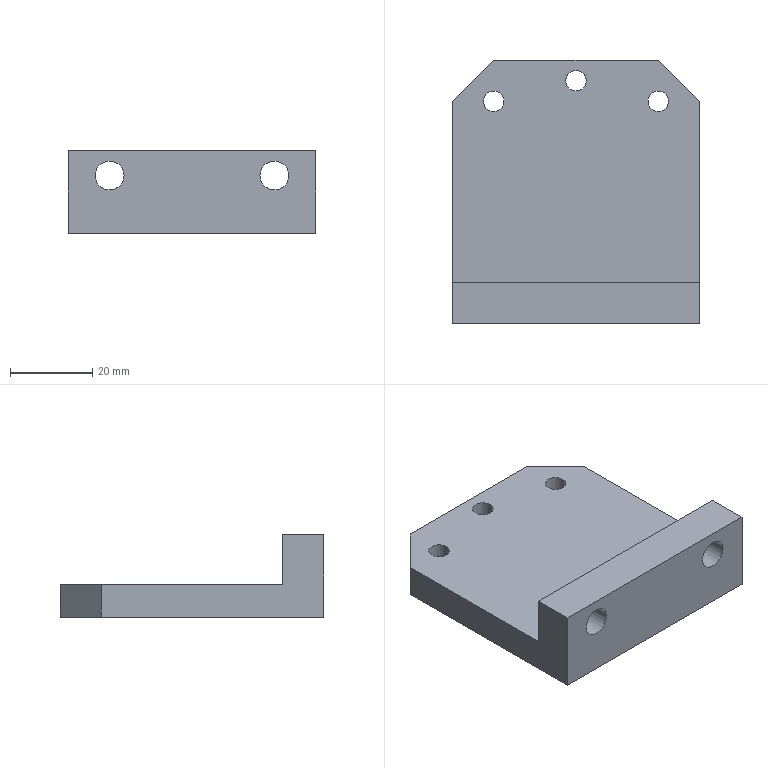Component | SolidWorks | STB-08-011-2 | 1 solid | 20 faces | box 60 x 64 x 20 mm | volume 35879 mm3 | cylinder 10 | plane 10 | commonest cylinder face diameters 5 x6 7 x4
build123d program:
from build123d import *

# Parameters (mm, degrees)
SKETCH1_W                = 20
SKETCH1_H                = 64
BOSS_EXTRUDE1_DEPTH      = 30
CUT_EXTRUDE1_REACH       = 70.731
SKETCH2_W                = 12
SKETCH2_H                = 54
M6_TAPPED_HOLE1_D        = 5
M6_TAPPED_HOLE2_D        = 5
M6_TAPPED_HOLE2_DEPTH    = 17
M6_TAPPED_HOLE2_TIP      = 1.502
CHAMFER1_SIZE            = 10
F_7_0_7_DIAMETER_HOLE1_D = 7


with BuildPart() as part:
    # Sketch1 → Boss-Extrude1 (new, symmetric)
    with BuildSketch(Plane.XY):
        Rectangle(SKETCH1_W, SKETCH1_H)
    extrude(amount=BOSS_EXTRUDE1_DEPTH, both=True)

    # Sketch2 → Cut-Extrude1 (cut, up to next)
    with BuildSketch(Plane.XY.offset(30), mode=Mode.PRIVATE) as cut_extrude1_sk1:
        with Locations((4, 5)):
            Rectangle(SKETCH2_W, SKETCH2_H)
    cut_extrude1_tool1 = extrude(cut_extrude1_sk1.sketch, amount=-CUT_EXTRUDE1_REACH, mode=Mode.PRIVATE) & part.part
    add(cut_extrude1_tool1.solids().sort_by_distance((4, 5, 30))[0], mode=Mode.SUBTRACT)

    # M6 Tapped Hole1 (through all)
    with Locations(Plane.ZY.offset(10)):
        with Locations((0, 27)):
            Hole(M6_TAPPED_HOLE1_D / 2)

    # M6 Tapped Hole2
    with Locations(Plane(origin=(-2, 0, 0), x_dir=(0, 0, -1), z_dir=(1, 0, 0))):
        with Locations((-20, 22), (20, 22)):
            Hole(M6_TAPPED_HOLE2_D / 2, depth=M6_TAPPED_HOLE2_DEPTH)
            with Locations((0, 0, -(M6_TAPPED_HOLE2_DEPTH + M6_TAPPED_HOLE2_TIP / 2))):  # 118° drill point
                Cone(0, M6_TAPPED_HOLE2_D / 2, M6_TAPPED_HOLE2_TIP, mode=Mode.SUBTRACT)

    # Chamfer1
    chamfer1_edges = [part.edges().sort_by_distance(p)[0] for p in [
        (-6, 32, -30),
        (-6, 32, 30),
    ]]
    chamfer(chamfer1_edges, length=CHAMFER1_SIZE)

    # 7.0 _7_ Diameter Hole1 (through all)
    with Locations(Plane(origin=(0, -22, 0), x_dir=(-1, 0, 0), z_dir=(0, 1, 0))):
        with Locations((-4, -20), (-4, 20)):
            Hole(F_7_0_7_DIAMETER_HOLE1_D / 2)


solid = part.part

# Placed as in the assembly
solid = solid.moved(Location((-104.904, 187.999, 11), (0, -90, 0)))
STEP:
#1=COLOUR_RGB('',0.7922,0.8196,0.9333);
#2=FILL_AREA_STYLE_COLOUR('',#1);
#3=FILL_AREA_STYLE('',(#2));
#4=SURFACE_STYLE_FILL_AREA(#3);
#5=SURFACE_SIDE_STYLE('',(#4));
#6=SURFACE_STYLE_USAGE(.BOTH.,#5);
#7=PRESENTATION_STYLE_ASSIGNMENT((#6));
#8=CARTESIAN_POINT('',(-3.205,6.142,0.5906));
#9=VERTEX_POINT('',#8);
#10=CARTESIAN_POINT('',(-3.48,6.142,0.5906));
#11=VERTEX_POINT('',#10);
#12=CARTESIAN_POINT('',(-3.343,6.142,0.5906));
#13=DIRECTION('',(-0.,1.,0.));
#14=DIRECTION('',(-1.,0.,0.));
#15=AXIS2_PLACEMENT_3D('',#12,#13,#14);
#16=CIRCLE('',#15,0.1378);
#17=EDGE_CURVE('',#9,#11,#16,.T.);
#18=ORIENTED_EDGE('',*,*,#17,.F.);
#19=CARTESIAN_POINT('',(-3.205,6.535,0.5906));
#20=VERTEX_POINT('',#19);
#21=CARTESIAN_POINT('',(-3.205,6.535,0.5906));
#22=DIRECTION('',(-0.,1.,0.));
#23=VECTOR('',#22,39.37);
#24=LINE('',#21,#23);
#25=EDGE_CURVE('',#9,#20,#24,.T.);
#26=ORIENTED_EDGE('',*,*,#25,.T.);
#27=CARTESIAN_POINT('',(-3.48,6.535,0.5906));
#28=VERTEX_POINT('',#27);
#29=CARTESIAN_POINT('',(-3.343,6.535,0.5906));
#30=DIRECTION('',(-0.,1.,0.));
#31=DIRECTION('',(-1.,0.,0.));
#32=AXIS2_PLACEMENT_3D('',#29,#30,#31);
#33=CIRCLE('',#32,0.1378);
#34=EDGE_CURVE('',#20,#28,#33,.T.);
#35=ORIENTED_EDGE('',*,*,#34,.T.);
#36=CARTESIAN_POINT('',(-3.48,6.535,0.5906));
#37=DIRECTION('',(-0.,1.,0.));
#38=VECTOR('',#37,39.37);
#39=LINE('',#36,#38);
#40=EDGE_CURVE('',#11,#28,#39,.T.);
#41=ORIENTED_EDGE('',*,*,#40,.F.);
#42=EDGE_LOOP('',(#18,#26,#35,#41));
#43=FACE_OUTER_BOUND('',#42,.T.);
#44=CARTESIAN_POINT('',(-3.343,6.535,0.5906));
#45=DIRECTION('',(-0.,1.,0.));
#46=DIRECTION('',(-1.,0.,0.));
#47=AXIS2_PLACEMENT_3D('',#44,#45,#46);
#48=CYLINDRICAL_SURFACE('',#47,0.1378);
#49=ADVANCED_FACE('',(#43),#48,.F.);
#50=CARTESIAN_POINT('',(-4.78,6.142,0.5906));
#51=VERTEX_POINT('',#50);
#52=CARTESIAN_POINT('',(-5.055,6.142,0.5906));
#53=VERTEX_POINT('',#52);
#54=CARTESIAN_POINT('',(-4.917,6.142,0.5906));
#55=DIRECTION('',(-0.,1.,0.));
#56=DIRECTION('',(-1.,0.,0.));
#57=AXIS2_PLACEMENT_3D('',#54,#55,#56);
#58=CIRCLE('',#57,0.1378);
#59=EDGE_CURVE('',#51,#53,#58,.T.);
#60=ORIENTED_EDGE('',*,*,#59,.F.);
#61=CARTESIAN_POINT('',(-4.78,6.535,0.5906));
#62=VERTEX_POINT('',#61);
#63=CARTESIAN_POINT('',(-4.78,6.535,0.5906));
#64=DIRECTION('',(-0.,1.,0.));
#65=VECTOR('',#64,39.37);
#66=LINE('',#63,#65);
#67=EDGE_CURVE('',#51,#62,#66,.T.);
#68=ORIENTED_EDGE('',*,*,#67,.T.);
#69=CARTESIAN_POINT('',(-5.055,6.535,0.5906));
#70=VERTEX_POINT('',#69);
#71=CARTESIAN_POINT('',(-4.917,6.535,0.5906));
#72=DIRECTION('',(-0.,1.,0.));
#73=DIRECTION('',(-1.,0.,0.));
#74=AXIS2_PLACEMENT_3D('',#71,#72,#73);
#75=CIRCLE('',#74,0.1378);
#76=EDGE_CURVE('',#62,#70,#75,.T.);
#77=ORIENTED_EDGE('',*,*,#76,.T.);
#78=CARTESIAN_POINT('',(-5.055,6.535,0.5906));
#79=DIRECTION('',(-0.,1.,0.));
#80=VECTOR('',#79,39.37);
#81=LINE('',#78,#80);
#82=EDGE_CURVE('',#53,#70,#81,.T.);
#83=ORIENTED_EDGE('',*,*,#82,.F.);
#84=EDGE_LOOP('',(#60,#68,#77,#83));
#85=FACE_OUTER_BOUND('',#84,.T.);
#86=CARTESIAN_POINT('',(-4.917,6.535,0.5906));
#87=DIRECTION('',(-0.,1.,0.));
#88=DIRECTION('',(-1.,0.,0.));
#89=AXIS2_PLACEMENT_3D('',#86,#87,#88);
#90=CYLINDRICAL_SURFACE('',#89,0.1378);
#91=ADVANCED_FACE('',(#85),#90,.F.);
#92=CARTESIAN_POINT('',(-5.016,8.268,0.03937));
#93=VERTEX_POINT('',#92);
#94=CARTESIAN_POINT('',(-4.819,8.268,0.03937));
#95=VERTEX_POINT('',#94);
#96=CARTESIAN_POINT('',(-4.917,8.268,0.03937));
#97=DIRECTION('',(-0.,0.,1.));
#98=DIRECTION('',(1.,0.,0.));
#99=AXIS2_PLACEMENT_3D('',#96,#97,#98);
#100=CIRCLE('',#99,0.09843);
#101=EDGE_CURVE('',#93,#95,#100,.T.);
#102=ORIENTED_EDGE('',*,*,#101,.F.);
#103=CARTESIAN_POINT('',(-5.016,8.268,0.3543));
#104=VERTEX_POINT('',#103);
#105=CARTESIAN_POINT('',(-5.016,8.268,0.3543));
#106=DIRECTION('',(-0.,0.,1.));
#107=VECTOR('',#106,39.37);
#108=LINE('',#105,#107);
#109=EDGE_CURVE('',#93,#104,#108,.T.);
#110=ORIENTED_EDGE('',*,*,#109,.T.);
#111=CARTESIAN_POINT('',(-4.819,8.268,0.3543));
#112=VERTEX_POINT('',#111);
#113=CARTESIAN_POINT('',(-4.917,8.268,0.3543));
#114=DIRECTION('',(-0.,0.,1.));
#115=DIRECTION('',(1.,0.,0.));
#116=AXIS2_PLACEMENT_3D('',#113,#114,#115);
#117=CIRCLE('',#116,0.09843);
#118=EDGE_CURVE('',#104,#112,#117,.T.);
#119=ORIENTED_EDGE('',*,*,#118,.T.);
#120=CARTESIAN_POINT('',(-4.819,8.268,0.3543));
#121=DIRECTION('',(-0.,0.,1.));
#122=VECTOR('',#121,39.37);
#123=LINE('',#120,#122);
#124=EDGE_CURVE('',#95,#112,#123,.T.);
#125=ORIENTED_EDGE('',*,*,#124,.F.);
#126=EDGE_LOOP('',(#102,#110,#119,#125));
#127=FACE_OUTER_BOUND('',#126,.T.);
#128=CARTESIAN_POINT('',(-4.917,8.268,0.3543));
#129=DIRECTION('',(-0.,0.,1.));
#130=DIRECTION('',(1.,0.,0.));
#131=AXIS2_PLACEMENT_3D('',#128,#129,#130);
#132=CYLINDRICAL_SURFACE('',#131,0.09843);
#133=ADVANCED_FACE('',(#127),#132,.F.);
#134=CARTESIAN_POINT('',(-3.441,8.268,0.03937));
#135=VERTEX_POINT('',#134);
#136=CARTESIAN_POINT('',(-3.244,8.268,0.03937));
#137=VERTEX_POINT('',#136);
#138=CARTESIAN_POINT('',(-3.343,8.268,0.03937));
#139=DIRECTION('',(-0.,0.,1.));
#140=DIRECTION('',(1.,0.,0.));
#141=AXIS2_PLACEMENT_3D('',#138,#139,#140);
#142=CIRCLE('',#141,0.09843);
#143=EDGE_CURVE('',#135,#137,#142,.T.);
#144=ORIENTED_EDGE('',*,*,#143,.F.);
#145=CARTESIAN_POINT('',(-3.441,8.268,0.3543));
#146=VERTEX_POINT('',#145);
#147=CARTESIAN_POINT('',(-3.441,8.268,0.3543));
#148=DIRECTION('',(-0.,0.,1.));
#149=VECTOR('',#148,39.37);
#150=LINE('',#147,#149);
#151=EDGE_CURVE('',#135,#146,#150,.T.);
#152=ORIENTED_EDGE('',*,*,#151,.T.);
#153=CARTESIAN_POINT('',(-3.244,8.268,0.3543));
#154=VERTEX_POINT('',#153);
#155=CARTESIAN_POINT('',(-3.343,8.268,0.3543));
#156=DIRECTION('',(-0.,0.,1.));
#157=DIRECTION('',(1.,0.,0.));
#158=AXIS2_PLACEMENT_3D('',#155,#156,#157);
#159=CIRCLE('',#158,0.09843);
#160=EDGE_CURVE('',#146,#154,#159,.T.);
#161=ORIENTED_EDGE('',*,*,#160,.T.);
#162=CARTESIAN_POINT('',(-3.244,8.268,0.3543));
#163=DIRECTION('',(-0.,0.,1.));
#164=VECTOR('',#163,39.37);
#165=LINE('',#162,#164);
#166=EDGE_CURVE('',#137,#154,#165,.T.);
#167=ORIENTED_EDGE('',*,*,#166,.F.);
#168=EDGE_LOOP('',(#144,#152,#161,#167));
#169=FACE_OUTER_BOUND('',#168,.T.);
#170=CARTESIAN_POINT('',(-3.343,8.268,0.3543));
#171=DIRECTION('',(-0.,0.,1.));
#172=DIRECTION('',(1.,0.,0.));
#173=AXIS2_PLACEMENT_3D('',#170,#171,#172);
#174=CYLINDRICAL_SURFACE('',#173,0.09843);
#175=ADVANCED_FACE('',(#169),#174,.F.);
#176=CARTESIAN_POINT('',(-4.032,8.465,0.3543));
#177=VERTEX_POINT('',#176);
#178=CARTESIAN_POINT('',(-4.228,8.465,0.3543));
#179=VERTEX_POINT('',#178);
#180=CARTESIAN_POINT('',(-4.13,8.465,0.3543));
#181=DIRECTION('',(0.,-0.,-1.));
#182=DIRECTION('',(0.,-1.,0.));
#183=AXIS2_PLACEMENT_3D('',#180,#181,#182);
#184=CIRCLE('',#183,0.09843);
#185=EDGE_CURVE('',#177,#179,#184,.T.);
#186=ORIENTED_EDGE('',*,*,#185,.F.);
#187=CARTESIAN_POINT('',(-4.032,8.465,0.03937));
#188=VERTEX_POINT('',#187);
#189=CARTESIAN_POINT('',(-4.032,8.465,0.03937));
#190=DIRECTION('',(0.,-0.,-1.));
#191=VECTOR('',#190,39.37);
#192=LINE('',#189,#191);
#193=EDGE_CURVE('',#177,#188,#192,.T.);
#194=ORIENTED_EDGE('',*,*,#193,.T.);
#195=CARTESIAN_POINT('',(-4.228,8.465,0.03937));
#196=VERTEX_POINT('',#195);
#197=CARTESIAN_POINT('',(-4.13,8.465,0.03937));
#198=DIRECTION('',(0.,-0.,-1.));
#199=DIRECTION('',(-1.,0.,-0.));
#200=AXIS2_PLACEMENT_3D('',#197,#198,#199);
#201=CIRCLE('',#200,0.09843);
#202=EDGE_CURVE('',#188,#196,#201,.T.);
#203=ORIENTED_EDGE('',*,*,#202,.T.);
#204=CARTESIAN_POINT('',(-4.228,8.465,0.03937));
#205=DIRECTION('',(0.,-0.,-1.));
#206=VECTOR('',#205,39.37);
#207=LINE('',#204,#206);
#208=EDGE_CURVE('',#179,#196,#207,.T.);
#209=ORIENTED_EDGE('',*,*,#208,.F.);
#210=EDGE_LOOP('',(#186,#194,#203,#209));
#211=FACE_OUTER_BOUND('',#210,.T.);
#212=CARTESIAN_POINT('',(-4.13,8.465,0.03937));
#213=DIRECTION('',(0.,-0.,-1.));
#214=DIRECTION('',(-1.,0.,-0.));
#215=AXIS2_PLACEMENT_3D('',#212,#213,#214);
#216=CYLINDRICAL_SURFACE('',#215,0.09843);
#217=ADVANCED_FACE('',(#211),#216,.F.);
#218=CARTESIAN_POINT('',(-4.13,8.465,0.3543));
#219=DIRECTION('',(0.,-0.,-1.));
#220=DIRECTION('',(0.,-1.,0.));
#221=AXIS2_PLACEMENT_3D('',#218,#219,#220);
#222=CIRCLE('',#221,0.09843);
#223=EDGE_CURVE('',#179,#177,#222,.T.);
#224=ORIENTED_EDGE('',*,*,#223,.T.);
#225=ORIENTED_EDGE('',*,*,#185,.T.);
#226=EDGE_LOOP('',(#224,#225));
#227=FACE_BOUND('',#226,.T.);
#228=CARTESIAN_POINT('',(-2.949,6.535,0.3543));
#229=VERTEX_POINT('',#228);
#230=CARTESIAN_POINT('',(-2.949,8.268,0.3543));
#231=VERTEX_POINT('',#230);
#232=CARTESIAN_POINT('',(-2.949,8.661,0.3543));
#233=DIRECTION('',(-0.,1.,-0.));
#234=VECTOR('',#233,39.37);
#235=LINE('',#232,#234);
#236=EDGE_CURVE('',#229,#231,#235,.T.);
#237=ORIENTED_EDGE('',*,*,#236,.T.);
#238=CARTESIAN_POINT('',(-3.343,8.661,0.3543));
#239=VERTEX_POINT('',#238);
#240=CARTESIAN_POINT('',(-3.343,8.661,0.3543));
#241=DIRECTION('',(-0.7071,0.7071,-0.));
#242=VECTOR('',#241,39.37);
#243=LINE('',#240,#242);
#244=EDGE_CURVE('',#231,#239,#243,.T.);
#245=ORIENTED_EDGE('',*,*,#244,.T.);
#246=CARTESIAN_POINT('',(-4.917,8.661,0.3543));
#247=VERTEX_POINT('',#246);
#248=CARTESIAN_POINT('',(-2.949,8.661,0.3543));
#249=DIRECTION('',(-1.,0.,-0.));
#250=VECTOR('',#249,39.37);
#251=LINE('',#248,#250);
#252=EDGE_CURVE('',#239,#247,#251,.T.);
#253=ORIENTED_EDGE('',*,*,#252,.T.);
#254=CARTESIAN_POINT('',(-5.311,8.268,0.3543));
#255=VERTEX_POINT('',#254);
#256=CARTESIAN_POINT('',(-5.311,8.268,0.3543));
#257=DIRECTION('',(-0.7071,-0.7071,-0.));
#258=VECTOR('',#257,39.37);
#259=LINE('',#256,#258);
#260=EDGE_CURVE('',#247,#255,#259,.T.);
#261=ORIENTED_EDGE('',*,*,#260,.T.);
#262=CARTESIAN_POINT('',(-5.311,6.535,0.3543));
#263=VERTEX_POINT('',#262);
#264=CARTESIAN_POINT('',(-5.311,8.661,0.3543));
#265=DIRECTION('',(0.,-1.,0.));
#266=VECTOR('',#265,39.37);
#267=LINE('',#264,#266);
#268=EDGE_CURVE('',#255,#263,#267,.T.);
#269=ORIENTED_EDGE('',*,*,#268,.T.);
#270=CARTESIAN_POINT('',(-2.949,6.535,0.3543));
#271=DIRECTION('',(-1.,0.,-0.));
#272=VECTOR('',#271,39.37);
#273=LINE('',#270,#272);
#274=EDGE_CURVE('',#229,#263,#273,.T.);
#275=ORIENTED_EDGE('',*,*,#274,.F.);
#276=EDGE_LOOP('',(#237,#245,#253,#261,#269,#275));
#277=FACE_OUTER_BOUND('',#276,.T.);
#278=CARTESIAN_POINT('',(-3.343,8.268,0.3543));
#279=DIRECTION('',(-0.,0.,1.));
#280=DIRECTION('',(1.,0.,0.));
#281=AXIS2_PLACEMENT_3D('',#278,#279,#280);
#282=CIRCLE('',#281,0.09843);
#283=EDGE_CURVE('',#154,#146,#282,.T.);
#284=ORIENTED_EDGE('',*,*,#283,.F.);
#285=ORIENTED_EDGE('',*,*,#160,.F.);
#286=EDGE_LOOP('',(#284,#285));
#287=FACE_BOUND('',#286,.T.);
#288=CARTESIAN_POINT('',(-4.917,8.268,0.3543));
#289=DIRECTION('',(-0.,0.,1.));
#290=DIRECTION('',(1.,0.,0.));
#291=AXIS2_PLACEMENT_3D('',#288,#289,#290);
#292=CIRCLE('',#291,0.09843);
#293=EDGE_CURVE('',#112,#104,#292,.T.);
#294=ORIENTED_EDGE('',*,*,#293,.F.);
#295=ORIENTED_EDGE('',*,*,#118,.F.);
#296=EDGE_LOOP('',(#294,#295));
#297=FACE_BOUND('',#296,.T.);
#298=CARTESIAN_POINT('',(-2.949,8.661,0.3543));
#299=DIRECTION('',(0.,-0.,-1.));
#300=DIRECTION('',(0.,-1.,0.));
#301=AXIS2_PLACEMENT_3D('',#298,#299,#300);
#302=PLANE('',#301);
#303=ADVANCED_FACE('',(#227,#277,#287,#297),#302,.F.);
#304=CARTESIAN_POINT('',(-4.917,8.268,0.03937));
#305=DIRECTION('',(-0.,0.,1.));
#306=DIRECTION('',(1.,0.,0.));
#307=AXIS2_PLACEMENT_3D('',#304,#305,#306);
#308=CIRCLE('',#307,0.09843);
#309=EDGE_CURVE('',#95,#93,#308,.T.);
#310=ORIENTED_EDGE('',*,*,#309,.T.);
#311=ORIENTED_EDGE('',*,*,#101,.T.);
#312=EDGE_LOOP('',(#310,#311));
#313=FACE_BOUND('',#312,.T.);
#314=CARTESIAN_POINT('',(-3.343,8.268,0.03937));
#315=DIRECTION('',(-0.,0.,1.));
#316=DIRECTION('',(1.,0.,0.));
#317=AXIS2_PLACEMENT_3D('',#314,#315,#316);
#318=CIRCLE('',#317,0.09843);
#319=EDGE_CURVE('',#137,#135,#318,.T.);
#320=ORIENTED_EDGE('',*,*,#319,.T.);
#321=ORIENTED_EDGE('',*,*,#143,.T.);
#322=EDGE_LOOP('',(#320,#321));
#323=FACE_BOUND('',#322,.T.);
#324=CARTESIAN_POINT('',(-4.13,8.465,0.03937));
#325=DIRECTION('',(0.,-0.,-1.));
#326=DIRECTION('',(-1.,0.,-0.));
#327=AXIS2_PLACEMENT_3D('',#324,#325,#326);
#328=CIRCLE('',#327,0.09843);
#329=EDGE_CURVE('',#196,#188,#328,.T.);
#330=ORIENTED_EDGE('',*,*,#329,.F.);
#331=ORIENTED_EDGE('',*,*,#202,.F.);
#332=EDGE_LOOP('',(#330,#331));
#333=FACE_BOUND('',#332,.T.);
#334=CARTESIAN_POINT('',(-4.917,8.661,0.03937));
#335=VERTEX_POINT('',#334);
#336=CARTESIAN_POINT('',(-3.343,8.661,0.03937));
#337=VERTEX_POINT('',#336);
#338=CARTESIAN_POINT('',(-5.311,8.661,0.03937));
#339=DIRECTION('',(1.,-0.,0.));
#340=VECTOR('',#339,39.37);
#341=LINE('',#338,#340);
#342=EDGE_CURVE('',#335,#337,#341,.T.);
#343=ORIENTED_EDGE('',*,*,#342,.T.);
#344=CARTESIAN_POINT('',(-2.949,8.268,0.03937));
#345=VERTEX_POINT('',#344);
#346=CARTESIAN_POINT('',(-3.343,8.661,0.03937));
#347=DIRECTION('',(0.7071,-0.7071,0.));
#348=VECTOR('',#347,39.37);
#349=LINE('',#346,#348);
#350=EDGE_CURVE('',#337,#345,#349,.T.);
#351=ORIENTED_EDGE('',*,*,#350,.T.);
#352=CARTESIAN_POINT('',(-2.949,6.142,0.03937));
#353=VERTEX_POINT('',#352);
#354=CARTESIAN_POINT('',(-2.949,8.661,0.03937));
#355=DIRECTION('',(0.,-1.,-0.));
#356=VECTOR('',#355,39.37);
#357=LINE('',#354,#356);
#358=EDGE_CURVE('',#345,#353,#357,.T.);
#359=ORIENTED_EDGE('',*,*,#358,.T.);
#360=CARTESIAN_POINT('',(-5.311,6.142,0.03937));
#361=VERTEX_POINT('',#360);
#362=CARTESIAN_POINT('',(-5.311,6.142,0.03937));
#363=DIRECTION('',(1.,-0.,0.));
#364=VECTOR('',#363,39.37);
#365=LINE('',#362,#364);
#366=EDGE_CURVE('',#361,#353,#365,.T.);
#367=ORIENTED_EDGE('',*,*,#366,.F.);
#368=CARTESIAN_POINT('',(-5.311,8.268,0.03937));
#369=VERTEX_POINT('',#368);
#370=CARTESIAN_POINT('',(-5.311,8.661,0.03937));
#371=DIRECTION('',(0.,-1.,-0.));
#372=VECTOR('',#371,39.37);
#373=LINE('',#370,#372);
#374=EDGE_CURVE('',#369,#361,#373,.T.);
#375=ORIENTED_EDGE('',*,*,#374,.F.);
#376=CARTESIAN_POINT('',(-5.311,8.268,0.03937));
#377=DIRECTION('',(0.7071,0.7071,0.));
#378=VECTOR('',#377,39.37);
#379=LINE('',#376,#378);
#380=EDGE_CURVE('',#369,#335,#379,.T.);
#381=ORIENTED_EDGE('',*,*,#380,.T.);
#382=EDGE_LOOP('',(#343,#351,#359,#367,#375,#381));
#383=FACE_OUTER_BOUND('',#382,.T.);
#384=CARTESIAN_POINT('',(-5.311,8.661,0.03937));
#385=DIRECTION('',(-0.,0.,1.));
#386=DIRECTION('',(1.,-0.,0.));
#387=AXIS2_PLACEMENT_3D('',#384,#385,#386);
#388=PLANE('',#387);
#389=ADVANCED_FACE('',(#313,#323,#333,#383),#388,.F.);
#390=CARTESIAN_POINT('',(-3.343,6.142,0.5906));
#391=DIRECTION('',(-0.,1.,0.));
#392=DIRECTION('',(-1.,0.,0.));
#393=AXIS2_PLACEMENT_3D('',#390,#391,#392);
#394=CIRCLE('',#393,0.1378);
#395=EDGE_CURVE('',#11,#9,#394,.T.);
#396=ORIENTED_EDGE('',*,*,#395,.T.);
#397=ORIENTED_EDGE('',*,*,#17,.T.);
#398=EDGE_LOOP('',(#396,#397));
#399=FACE_BOUND('',#398,.T.);
#400=CARTESIAN_POINT('',(-4.917,6.142,0.5906));
#401=DIRECTION('',(-0.,1.,0.));
#402=DIRECTION('',(-1.,0.,0.));
#403=AXIS2_PLACEMENT_3D('',#400,#401,#402);
#404=CIRCLE('',#403,0.1378);
#405=EDGE_CURVE('',#53,#51,#404,.T.);
#406=ORIENTED_EDGE('',*,*,#405,.T.);
#407=ORIENTED_EDGE('',*,*,#59,.T.);
#408=EDGE_LOOP('',(#406,#407));
#409=FACE_BOUND('',#408,.T.);
#410=CARTESIAN_POINT('',(-2.949,6.142,0.8268));
#411=VERTEX_POINT('',#410);
#412=CARTESIAN_POINT('',(-2.949,6.142,0.03937));
#413=DIRECTION('',(-0.,0.,1.));
#414=VECTOR('',#413,39.37);
#415=LINE('',#412,#414);
#416=EDGE_CURVE('',#353,#411,#415,.T.);
#417=ORIENTED_EDGE('',*,*,#416,.T.);
#418=CARTESIAN_POINT('',(-5.311,6.142,0.8268));
#419=VERTEX_POINT('',#418);
#420=CARTESIAN_POINT('',(-5.311,6.142,0.8268));
#421=DIRECTION('',(1.,-0.,0.));
#422=VECTOR('',#421,39.37);
#423=LINE('',#420,#422);
#424=EDGE_CURVE('',#419,#411,#423,.T.);
#425=ORIENTED_EDGE('',*,*,#424,.F.);
#426=CARTESIAN_POINT('',(-5.311,6.142,0.03937));
#427=DIRECTION('',(-0.,0.,1.));
#428=VECTOR('',#427,39.37);
#429=LINE('',#426,#428);
#430=EDGE_CURVE('',#361,#419,#429,.T.);
#431=ORIENTED_EDGE('',*,*,#430,.F.);
#432=ORIENTED_EDGE('',*,*,#366,.T.);
#433=EDGE_LOOP('',(#417,#425,#431,#432));
#434=FACE_OUTER_BOUND('',#433,.T.);
#435=CARTESIAN_POINT('',(-5.311,6.142,0.03937));
#436=DIRECTION('',(0.,1.,0.));
#437=DIRECTION('',(-1.,0.,-0.));
#438=AXIS2_PLACEMENT_3D('',#435,#436,#437);
#439=PLANE('',#438);
#440=ADVANCED_FACE('',(#399,#409,#434),#439,.F.);
#441=CARTESIAN_POINT('',(-2.949,6.535,0.8268));
#442=VERTEX_POINT('',#441);
#443=CARTESIAN_POINT('',(-2.949,8.661,0.8268));
#444=DIRECTION('',(-0.,1.,0.));
#445=VECTOR('',#444,39.37);
#446=LINE('',#443,#445);
#447=EDGE_CURVE('',#411,#442,#446,.T.);
#448=ORIENTED_EDGE('',*,*,#447,.T.);
#449=CARTESIAN_POINT('',(-5.311,6.535,0.8268));
#450=VERTEX_POINT('',#449);
#451=CARTESIAN_POINT('',(-2.949,6.535,0.8268));
#452=DIRECTION('',(-1.,0.,-0.));
#453=VECTOR('',#452,39.37);
#454=LINE('',#451,#453);
#455=EDGE_CURVE('',#442,#450,#454,.T.);
#456=ORIENTED_EDGE('',*,*,#455,.T.);
#457=CARTESIAN_POINT('',(-5.311,8.661,0.8268));
#458=DIRECTION('',(-0.,1.,0.));
#459=VECTOR('',#458,39.37);
#460=LINE('',#457,#459);
#461=EDGE_CURVE('',#419,#450,#460,.T.);
#462=ORIENTED_EDGE('',*,*,#461,.F.);
#463=ORIENTED_EDGE('',*,*,#424,.T.);
#464=EDGE_LOOP('',(#448,#456,#462,#463));
#465=FACE_OUTER_BOUND('',#464,.T.);
#466=CARTESIAN_POINT('',(-5.311,8.661,0.8268));
#467=DIRECTION('',(0.,-0.,-1.));
#468=DIRECTION('',(-1.,0.,-0.));
#469=AXIS2_PLACEMENT_3D('',#466,#467,#468);
#470=PLANE('',#469);
#471=ADVANCED_FACE('',(#465),#470,.F.);
#472=ORIENTED_EDGE('',*,*,#252,.F.);
#473=CARTESIAN_POINT('',(-3.343,8.661,0.03937));
#474=DIRECTION('',(0.,-0.,-1.));
#475=VECTOR('',#474,39.37);
#476=LINE('',#473,#475);
#477=EDGE_CURVE('',#239,#337,#476,.T.);
#478=ORIENTED_EDGE('',*,*,#477,.T.);
#479=ORIENTED_EDGE('',*,*,#342,.F.);
#480=CARTESIAN_POINT('',(-4.917,8.661,0.3543));
#481=DIRECTION('',(-0.,0.,1.));
#482=VECTOR('',#481,39.37);
#483=LINE('',#480,#482);
#484=EDGE_CURVE('',#335,#247,#483,.T.);
#485=ORIENTED_EDGE('',*,*,#484,.T.);
#486=EDGE_LOOP('',(#472,#478,#479,#485));
#487=FACE_OUTER_BOUND('',#486,.T.);
#488=CARTESIAN_POINT('',(-5.311,8.661,0.03937));
#489=DIRECTION('',(-0.,-1.,-0.));
#490=DIRECTION('',(1.,-0.,0.));
#491=AXIS2_PLACEMENT_3D('',#488,#489,#490);
#492=PLANE('',#491);
#493=ADVANCED_FACE('',(#487),#492,.F.);
#494=ORIENTED_EDGE('',*,*,#268,.F.);
#495=CARTESIAN_POINT('',(-5.311,8.268,0.03937));
#496=DIRECTION('',(0.,-0.,-1.));
#497=VECTOR('',#496,39.37);
#498=LINE('',#495,#497);
#499=EDGE_CURVE('',#255,#369,#498,.T.);
#500=ORIENTED_EDGE('',*,*,#499,.T.);
#501=ORIENTED_EDGE('',*,*,#374,.T.);
#502=ORIENTED_EDGE('',*,*,#430,.T.);
#503=ORIENTED_EDGE('',*,*,#461,.T.);
#504=CARTESIAN_POINT('',(-5.311,6.535,0.8268));
#505=DIRECTION('',(-0.,0.,1.));
#506=VECTOR('',#505,39.37);
#507=LINE('',#504,#506);
#508=EDGE_CURVE('',#263,#450,#507,.T.);
#509=ORIENTED_EDGE('',*,*,#508,.F.);
#510=EDGE_LOOP('',(#494,#500,#501,#502,#503,#509));
#511=FACE_OUTER_BOUND('',#510,.T.);
#512=CARTESIAN_POINT('',(-5.311,6.142,0.03937));
#513=DIRECTION('',(-1.,0.,-0.));
#514=DIRECTION('',(-0.,0.,1.));
#515=AXIS2_PLACEMENT_3D('',#512,#513,#514);
#516=PLANE('',#515);
#517=ADVANCED_FACE('',(#511),#516,.T.);
#518=ORIENTED_EDGE('',*,*,#358,.F.);
#519=CARTESIAN_POINT('',(-2.949,8.268,0.03937));
#520=DIRECTION('',(-0.,0.,1.));
#521=VECTOR('',#520,39.37);
#522=LINE('',#519,#521);
#523=EDGE_CURVE('',#345,#231,#522,.T.);
#524=ORIENTED_EDGE('',*,*,#523,.T.);
#525=ORIENTED_EDGE('',*,*,#236,.F.);
#526=CARTESIAN_POINT('',(-2.949,6.535,0.8268));
#527=DIRECTION('',(0.,-0.,-1.));
#528=VECTOR('',#527,39.37);
#529=LINE('',#526,#528);
#530=EDGE_CURVE('',#442,#229,#529,.T.);
#531=ORIENTED_EDGE('',*,*,#530,.F.);
#532=ORIENTED_EDGE('',*,*,#447,.F.);
#533=ORIENTED_EDGE('',*,*,#416,.F.);
#534=EDGE_LOOP('',(#518,#524,#525,#531,#532,#533));
#535=FACE_OUTER_BOUND('',#534,.T.);
#536=CARTESIAN_POINT('',(-2.949,6.142,0.03937));
#537=DIRECTION('',(-1.,0.,-0.));
#538=DIRECTION('',(-0.,0.,1.));
#539=AXIS2_PLACEMENT_3D('',#536,#537,#538);
#540=PLANE('',#539);
#541=ADVANCED_FACE('',(#535),#540,.F.);
#542=CARTESIAN_POINT('',(-3.343,6.535,0.5906));
#543=DIRECTION('',(-0.,1.,0.));
#544=DIRECTION('',(-1.,0.,0.));
#545=AXIS2_PLACEMENT_3D('',#542,#543,#544);
#546=CIRCLE('',#545,0.1378);
#547=EDGE_CURVE('',#28,#20,#546,.T.);
#548=ORIENTED_EDGE('',*,*,#547,.F.);
#549=ORIENTED_EDGE('',*,*,#34,.F.);
#550=EDGE_LOOP('',(#548,#549));
#551=FACE_BOUND('',#550,.T.);
#552=CARTESIAN_POINT('',(-4.917,6.535,0.5906));
#553=DIRECTION('',(-0.,1.,0.));
#554=DIRECTION('',(-1.,0.,0.));
#555=AXIS2_PLACEMENT_3D('',#552,#553,#554);
#556=CIRCLE('',#555,0.1378);
#557=EDGE_CURVE('',#70,#62,#556,.T.);
#558=ORIENTED_EDGE('',*,*,#557,.F.);
#559=ORIENTED_EDGE('',*,*,#76,.F.);
#560=EDGE_LOOP('',(#558,#559));
#561=FACE_BOUND('',#560,.T.);
#562=ORIENTED_EDGE('',*,*,#530,.T.);
#563=ORIENTED_EDGE('',*,*,#274,.T.);
#564=ORIENTED_EDGE('',*,*,#508,.T.);
#565=ORIENTED_EDGE('',*,*,#455,.F.);
#566=EDGE_LOOP('',(#562,#563,#564,#565));
#567=FACE_OUTER_BOUND('',#566,.T.);
#568=CARTESIAN_POINT('',(-2.949,6.535,0.8268));
#569=DIRECTION('',(-0.,-1.,-0.));
#570=DIRECTION('',(1.,-0.,0.));
#571=AXIS2_PLACEMENT_3D('',#568,#569,#570);
#572=PLANE('',#571);
#573=ADVANCED_FACE('',(#551,#561,#567),#572,.F.);
#574=ORIENTED_EDGE('',*,*,#193,.F.);
#575=ORIENTED_EDGE('',*,*,#223,.F.);
#576=ORIENTED_EDGE('',*,*,#208,.T.);
#577=ORIENTED_EDGE('',*,*,#329,.T.);
#578=EDGE_LOOP('',(#574,#575,#576,#577));
#579=FACE_OUTER_BOUND('',#578,.T.);
#580=CARTESIAN_POINT('',(-4.13,8.465,0.03937));
#581=DIRECTION('',(0.,-0.,-1.));
#582=DIRECTION('',(-1.,0.,-0.));
#583=AXIS2_PLACEMENT_3D('',#580,#581,#582);
#584=CYLINDRICAL_SURFACE('',#583,0.09843);
#585=ADVANCED_FACE('',(#579),#584,.F.);
#586=ORIENTED_EDGE('',*,*,#151,.F.);
#587=ORIENTED_EDGE('',*,*,#319,.F.);
#588=ORIENTED_EDGE('',*,*,#166,.T.);
#589=ORIENTED_EDGE('',*,*,#283,.T.);
#590=EDGE_LOOP('',(#586,#587,#588,#589));
#591=FACE_OUTER_BOUND('',#590,.T.);
#592=CARTESIAN_POINT('',(-3.343,8.268,0.3543));
#593=DIRECTION('',(-0.,0.,1.));
#594=DIRECTION('',(1.,0.,0.));
#595=AXIS2_PLACEMENT_3D('',#592,#593,#594);
#596=CYLINDRICAL_SURFACE('',#595,0.09843);
#597=ADVANCED_FACE('',(#591),#596,.F.);
#598=ORIENTED_EDGE('',*,*,#109,.F.);
#599=ORIENTED_EDGE('',*,*,#309,.F.);
#600=ORIENTED_EDGE('',*,*,#124,.T.);
#601=ORIENTED_EDGE('',*,*,#293,.T.);
#602=EDGE_LOOP('',(#598,#599,#600,#601));
#603=FACE_OUTER_BOUND('',#602,.T.);
#604=CARTESIAN_POINT('',(-4.917,8.268,0.3543));
#605=DIRECTION('',(-0.,0.,1.));
#606=DIRECTION('',(1.,0.,0.));
#607=AXIS2_PLACEMENT_3D('',#604,#605,#606);
#608=CYLINDRICAL_SURFACE('',#607,0.09843);
#609=ADVANCED_FACE('',(#603),#608,.F.);
#610=ORIENTED_EDGE('',*,*,#244,.F.);
#611=ORIENTED_EDGE('',*,*,#523,.F.);
#612=ORIENTED_EDGE('',*,*,#350,.F.);
#613=ORIENTED_EDGE('',*,*,#477,.F.);
#614=EDGE_LOOP('',(#610,#611,#612,#613));
#615=FACE_OUTER_BOUND('',#614,.T.);
#616=CARTESIAN_POINT('',(-3.343,8.661,0.03937));
#617=DIRECTION('',(-0.7071,-0.7071,-0.));
#618=DIRECTION('',(0.7071,-0.7071,0.));
#619=AXIS2_PLACEMENT_3D('',#616,#617,#618);
#620=PLANE('',#619);
#621=ADVANCED_FACE('',(#615),#620,.F.);
#622=ORIENTED_EDGE('',*,*,#260,.F.);
#623=ORIENTED_EDGE('',*,*,#484,.F.);
#624=ORIENTED_EDGE('',*,*,#380,.F.);
#625=ORIENTED_EDGE('',*,*,#499,.F.);
#626=EDGE_LOOP('',(#622,#623,#624,#625));
#627=FACE_OUTER_BOUND('',#626,.T.);
#628=CARTESIAN_POINT('',(-5.311,8.268,0.03937));
#629=DIRECTION('',(-0.7071,0.7071,-0.));
#630=DIRECTION('',(-0.7071,-0.7071,-0.));
#631=AXIS2_PLACEMENT_3D('',#628,#629,#630);
#632=PLANE('',#631);
#633=ADVANCED_FACE('',(#627),#632,.T.);
#634=ORIENTED_EDGE('',*,*,#67,.F.);
#635=ORIENTED_EDGE('',*,*,#405,.F.);
#636=ORIENTED_EDGE('',*,*,#82,.T.);
#637=ORIENTED_EDGE('',*,*,#557,.T.);
#638=EDGE_LOOP('',(#634,#635,#636,#637));
#639=FACE_OUTER_BOUND('',#638,.T.);
#640=CARTESIAN_POINT('',(-4.917,6.535,0.5906));
#641=DIRECTION('',(-0.,1.,0.));
#642=DIRECTION('',(-1.,0.,0.));
#643=AXIS2_PLACEMENT_3D('',#640,#641,#642);
#644=CYLINDRICAL_SURFACE('',#643,0.1378);
#645=ADVANCED_FACE('',(#639),#644,.F.);
#646=ORIENTED_EDGE('',*,*,#25,.F.);
#647=ORIENTED_EDGE('',*,*,#395,.F.);
#648=ORIENTED_EDGE('',*,*,#40,.T.);
#649=ORIENTED_EDGE('',*,*,#547,.T.);
#650=EDGE_LOOP('',(#646,#647,#648,#649));
#651=FACE_OUTER_BOUND('',#650,.T.);
#652=CARTESIAN_POINT('',(-3.343,6.535,0.5906));
#653=DIRECTION('',(-0.,1.,0.));
#654=DIRECTION('',(-1.,0.,0.));
#655=AXIS2_PLACEMENT_3D('',#652,#653,#654);
#656=CYLINDRICAL_SURFACE('',#655,0.1378);
#657=ADVANCED_FACE('',(#651),#656,.F.);
#658=CLOSED_SHELL('',(#49,#91,#133,#175,#217,#303,#389,#440,#471,#493,#517,#541,#573,#585,#597,#609,#621,#633,#645,#657));
#659=MANIFOLD_SOLID_BREP('',#658);
#660=STYLED_ITEM('',(#7),#659);
#661=(LENGTH_UNIT()NAMED_UNIT(*)SI_UNIT($,.METRE.));
#662=LENGTH_MEASURE_WITH_UNIT(LENGTH_MEASURE(0.0254),#661);
#663=DIMENSIONAL_EXPONENTS(1.,0.,0.,0.,0.,0.,0.);
#664=(CONVERSION_BASED_UNIT('',#662)LENGTH_UNIT()NAMED_UNIT(#663));
#665=UNCERTAINTY_MEASURE_WITH_UNIT(LENGTH_MEASURE(0.00001),#664,'','');
#666=(NAMED_UNIT(*)PLANE_ANGLE_UNIT()SI_UNIT($,.RADIAN.));
#667=(NAMED_UNIT(*)SI_UNIT($,.STERADIAN.)SOLID_ANGLE_UNIT());
#668=(GEOMETRIC_REPRESENTATION_CONTEXT(3)GLOBAL_UNCERTAINTY_ASSIGNED_CONTEXT((#665))GLOBAL_UNIT_ASSIGNED_CONTEXT((#664,#666,#667))REPRESENTATION_CONTEXT('',''));
#669=MECHANICAL_DESIGN_GEOMETRIC_PRESENTATION_REPRESENTATION('',(#660),#668);
#670=CARTESIAN_POINT('',(0.,0.,0.));
#671=DIRECTION('',(0.,0.,1.));
#672=DIRECTION('',(1.,0.,0.));
#673=AXIS2_PLACEMENT_3D('',#670,#671,#672);
#674=(LENGTH_UNIT()NAMED_UNIT(*)SI_UNIT($,.METRE.));
#675=LENGTH_MEASURE_WITH_UNIT(LENGTH_MEASURE(0.0254),#674);
#676=DIMENSIONAL_EXPONENTS(1.,0.,0.,0.,0.,0.,0.);
#677=(CONVERSION_BASED_UNIT('',#675)LENGTH_UNIT()NAMED_UNIT(#676));
#678=UNCERTAINTY_MEASURE_WITH_UNIT(LENGTH_MEASURE(0.00001),#677,'','');
#679=(NAMED_UNIT(*)PLANE_ANGLE_UNIT()SI_UNIT($,.RADIAN.));
#680=(NAMED_UNIT(*)SI_UNIT($,.STERADIAN.)SOLID_ANGLE_UNIT());
#681=(GEOMETRIC_REPRESENTATION_CONTEXT(3)GLOBAL_UNCERTAINTY_ASSIGNED_CONTEXT((#678))GLOBAL_UNIT_ASSIGNED_CONTEXT((#677,#679,#680))REPRESENTATION_CONTEXT('',''));
#682=ADVANCED_BREP_SHAPE_REPRESENTATION('',(#659,#673),#681);
#683=PRESENTATION_LAYER_ASSIGNMENT('','',(#660));